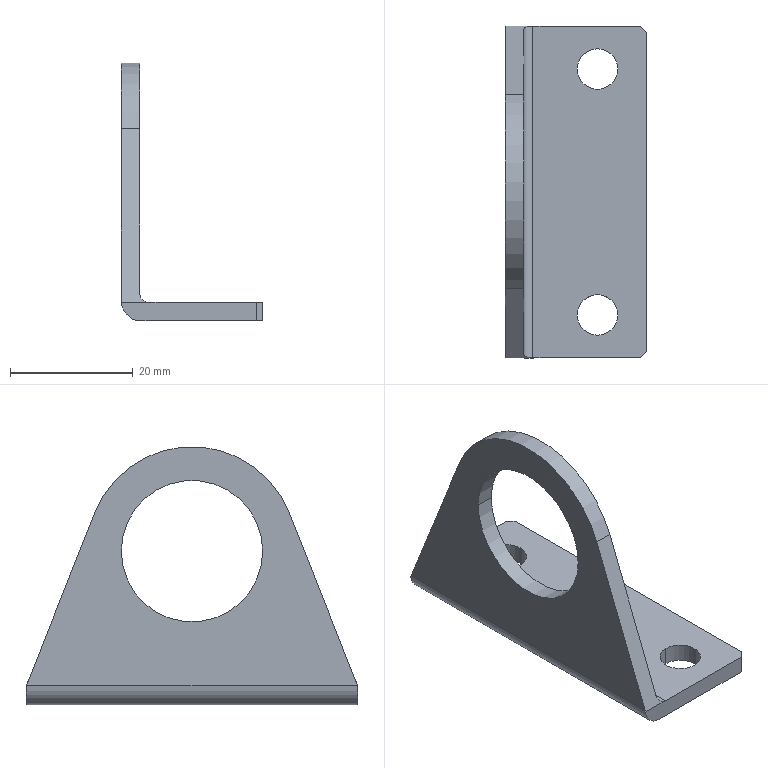Component | SolidWorks | CTM-HVS-42-02-27-1 | 1 solid | 20 faces | box 23 x 54 x 42 mm | volume 6546 mm3 | plane 11 | cylinder 9 | commonest cylinder face diameters 6.6 x4 23 x2 6.4 x1 3 x1 34 x1 | material Q235A Cold Rolled Sheet 3mm
build123d program:
from build123d import *

# Parameters (mm, degrees)
BOSS_EXTRUDE1_DEPTH      = 27
BOSS_EXTRUDE1_DEPTH_BACK = 27
CUT_EXTRUDE1_DEPTH       = 3
CUT_EXTRUDE1_DEPTH_BACK  = 3
SKETCH2_R                = 11.5
CUT_EXTRUDE2_DEPTH       = 6
CUT_EXTRUDE2_DEPTH_BACK  = 6
M6_CLEARANCE_HOLE1_D     = 6.6
CHAMFER1_SIZE            = 1


with BuildPart() as part:
    # Sketch1 → Boss-Extrude1 (new, two sides: drawn at the far end of the back side and taken through both)
    with BuildSketch(Plane.XY.offset(-BOSS_EXTRUDE1_DEPTH_BACK)):
        with BuildLine():
            Line((0, 17), (0, -21.8))
            ThreePointArc((0, -21.8), (0.9373, -24.063), (3.2, -25))
            Line((3.2, -25), (23, -25))
            Line((23, -25), (23, -22))
            Line((23, -22), (4.5, -22))
            ThreePointArc((4.5, -22), (3.439, -21.561), (3, -20.5))
            Line((3, -20.5), (3, 17))
            Line((3, 17), (0, 17))
        make_face()
    extrude(amount=BOSS_EXTRUDE1_DEPTH + BOSS_EXTRUDE1_DEPTH_BACK)

    # Sketch2 → Cut-Extrude1 (cut, two sides: drawn at the far end of the back side and taken through both)
    with BuildSketch(Plane(origin=(0, 0, 0), x_dir=(0, 0, -1), z_dir=(1, 0, 0)).offset(-CUT_EXTRUDE1_DEPTH_BACK)):
        Circle(SKETCH2_R)
    extrude(amount=CUT_EXTRUDE1_DEPTH + CUT_EXTRUDE1_DEPTH_BACK, mode=Mode.SUBTRACT)

    # Sketch3 → Cut-Extrude2 (cut, two sides: drawn at the far end of the back side and taken through both)
    with BuildSketch(Plane(origin=(0, 0, 0), x_dir=(0, 0, -1), z_dir=(1, 0, 0)).offset(-CUT_EXTRUDE2_DEPTH_BACK)):
        with BuildLine():
            Line((-44, -22), (-27, -22))
            Line((-27, -22), (-15.805, 6.261))
            ThreePointArc((-15.805, 6.261), (0, 17), (15.805, 6.261))
            Line((15.805, 6.261), (27, -22))
            Line((27, -22), (44, -22))
            Line((44, -22), (44, 59))
            Line((44, 59), (-44, 59))
            Line((-44, 59), (-44, -22))
        make_face()
    extrude(amount=CUT_EXTRUDE2_DEPTH + CUT_EXTRUDE2_DEPTH_BACK, mode=Mode.SUBTRACT)

    # M6 Clearance Hole1 (through all)
    with Locations(Plane(origin=(0, -22, 0), x_dir=(-1, 0, 0), z_dir=(0, 1, 0))):
        with Locations((-15, 20), (-15, -20)):
            Hole(M6_CLEARANCE_HOLE1_D / 2)

    # Chamfer1
    chamfer1_edges = [part.edges().sort_by_distance(p)[0] for p in [
        (23, -23.5, 27),
        (23, -23.5, -27),
    ]]
    chamfer(chamfer1_edges, length=CHAMFER1_SIZE)


solid = part.part

# Placed as in the assembly
solid = solid.moved(Location((-17.307, 55.443, 30), (90, 0, 0)))
STEP:
#1=CARTESIAN_POINT('',(-0.09084,1.525,0.1969));
#2=VERTEX_POINT('',#1);
#3=CARTESIAN_POINT('',(-0.09084,1.265,0.1969));
#4=VERTEX_POINT('',#3);
#5=CARTESIAN_POINT('',(-0.09084,1.395,0.1969));
#6=DIRECTION('',(0.,0.,1.));
#7=DIRECTION('',(0.,-1.,0.));
#8=AXIS2_PLACEMENT_3D('',#5,#6,#7);
#9=CIRCLE('',#8,0.1299);
#10=EDGE_CURVE('',#2,#4,#9,.T.);
#11=ORIENTED_EDGE('',*,*,#10,.F.);
#12=CARTESIAN_POINT('',(-0.09084,1.525,0.315));
#13=VERTEX_POINT('',#12);
#14=CARTESIAN_POINT('',(-0.09084,1.525,0.315));
#15=DIRECTION('',(0.,0.,1.));
#16=VECTOR('',#15,39.37);
#17=LINE('',#14,#16);
#18=EDGE_CURVE('',#2,#13,#17,.T.);
#19=ORIENTED_EDGE('',*,*,#18,.T.);
#20=CARTESIAN_POINT('',(-0.09084,1.265,0.315));
#21=VERTEX_POINT('',#20);
#22=CARTESIAN_POINT('',(-0.09084,1.395,0.315));
#23=DIRECTION('',(0.,0.,1.));
#24=DIRECTION('',(0.,-1.,0.));
#25=AXIS2_PLACEMENT_3D('',#22,#23,#24);
#26=CIRCLE('',#25,0.1299);
#27=EDGE_CURVE('',#13,#21,#26,.T.);
#28=ORIENTED_EDGE('',*,*,#27,.T.);
#29=CARTESIAN_POINT('',(-0.09084,1.265,0.315));
#30=DIRECTION('',(0.,0.,1.));
#31=VECTOR('',#30,39.37);
#32=LINE('',#29,#31);
#33=EDGE_CURVE('',#4,#21,#32,.T.);
#34=ORIENTED_EDGE('',*,*,#33,.F.);
#35=EDGE_LOOP('',(#11,#19,#28,#34));
#36=FACE_OUTER_BOUND('',#35,.T.);
#37=CARTESIAN_POINT('',(-0.09084,1.395,0.315));
#38=DIRECTION('',(0.,0.,1.));
#39=DIRECTION('',(0.,-1.,0.));
#40=AXIS2_PLACEMENT_3D('',#37,#38,#39);
#41=CYLINDRICAL_SURFACE('',#40,0.1299);
#42=ADVANCED_FACE('',(#36),#41,.F.);
#43=CARTESIAN_POINT('',(-0.09084,3.1,0.1969));
#44=VERTEX_POINT('',#43);
#45=CARTESIAN_POINT('',(-0.09084,2.84,0.1969));
#46=VERTEX_POINT('',#45);
#47=CARTESIAN_POINT('',(-0.09084,2.97,0.1969));
#48=DIRECTION('',(0.,0.,1.));
#49=DIRECTION('',(0.,-1.,0.));
#50=AXIS2_PLACEMENT_3D('',#47,#48,#49);
#51=CIRCLE('',#50,0.1299);
#52=EDGE_CURVE('',#44,#46,#51,.T.);
#53=ORIENTED_EDGE('',*,*,#52,.F.);
#54=CARTESIAN_POINT('',(-0.09084,3.1,0.315));
#55=VERTEX_POINT('',#54);
#56=CARTESIAN_POINT('',(-0.09084,3.1,0.315));
#57=DIRECTION('',(0.,0.,1.));
#58=VECTOR('',#57,39.37);
#59=LINE('',#56,#58);
#60=EDGE_CURVE('',#44,#55,#59,.T.);
#61=ORIENTED_EDGE('',*,*,#60,.T.);
#62=CARTESIAN_POINT('',(-0.09084,2.84,0.315));
#63=VERTEX_POINT('',#62);
#64=CARTESIAN_POINT('',(-0.09084,2.97,0.315));
#65=DIRECTION('',(0.,0.,1.));
#66=DIRECTION('',(0.,-1.,0.));
#67=AXIS2_PLACEMENT_3D('',#64,#65,#66);
#68=CIRCLE('',#67,0.1299);
#69=EDGE_CURVE('',#55,#63,#68,.T.);
#70=ORIENTED_EDGE('',*,*,#69,.T.);
#71=CARTESIAN_POINT('',(-0.09084,2.84,0.315));
#72=DIRECTION('',(0.,0.,1.));
#73=VECTOR('',#72,39.37);
#74=LINE('',#71,#73);
#75=EDGE_CURVE('',#46,#63,#74,.T.);
#76=ORIENTED_EDGE('',*,*,#75,.F.);
#77=EDGE_LOOP('',(#53,#61,#70,#76));
#78=FACE_OUTER_BOUND('',#77,.T.);
#79=CARTESIAN_POINT('',(-0.09084,2.97,0.315));
#80=DIRECTION('',(0.,0.,1.));
#81=DIRECTION('',(0.,-1.,0.));
#82=AXIS2_PLACEMENT_3D('',#79,#80,#81);
#83=CYLINDRICAL_SURFACE('',#82,0.1299);
#84=ADVANCED_FACE('',(#78),#83,.F.);
#85=CARTESIAN_POINT('',(-0.6814,1.73,1.181));
#86=VERTEX_POINT('',#85);
#87=CARTESIAN_POINT('',(-0.6814,2.636,1.181));
#88=VERTEX_POINT('',#87);
#89=CARTESIAN_POINT('',(-0.6814,2.183,1.181));
#90=DIRECTION('',(1.,0.,-0.));
#91=DIRECTION('',(-0.,1.,0.));
#92=AXIS2_PLACEMENT_3D('',#89,#90,#91);
#93=CIRCLE('',#92,0.4528);
#94=EDGE_CURVE('',#86,#88,#93,.T.);
#95=ORIENTED_EDGE('',*,*,#94,.F.);
#96=CARTESIAN_POINT('',(-0.5633,1.73,1.181));
#97=VERTEX_POINT('',#96);
#98=CARTESIAN_POINT('',(-0.7995,1.73,1.181));
#99=DIRECTION('',(1.,0.,-0.));
#100=VECTOR('',#99,39.37);
#101=LINE('',#98,#100);
#102=EDGE_CURVE('',#86,#97,#101,.T.);
#103=ORIENTED_EDGE('',*,*,#102,.T.);
#104=CARTESIAN_POINT('',(-0.5633,2.636,1.181));
#105=VERTEX_POINT('',#104);
#106=CARTESIAN_POINT('',(-0.5633,2.183,1.181));
#107=DIRECTION('',(1.,0.,-0.));
#108=DIRECTION('',(-0.,1.,0.));
#109=AXIS2_PLACEMENT_3D('',#106,#107,#108);
#110=CIRCLE('',#109,0.4528);
#111=EDGE_CURVE('',#97,#105,#110,.T.);
#112=ORIENTED_EDGE('',*,*,#111,.T.);
#113=CARTESIAN_POINT('',(-0.7995,2.636,1.181));
#114=DIRECTION('',(1.,0.,-0.));
#115=VECTOR('',#114,39.37);
#116=LINE('',#113,#115);
#117=EDGE_CURVE('',#88,#105,#116,.T.);
#118=ORIENTED_EDGE('',*,*,#117,.F.);
#119=EDGE_LOOP('',(#95,#103,#112,#118));
#120=FACE_OUTER_BOUND('',#119,.T.);
#121=CARTESIAN_POINT('',(-0.7995,2.183,1.181));
#122=DIRECTION('',(1.,0.,-0.));
#123=DIRECTION('',(-0.,1.,0.));
#124=AXIS2_PLACEMENT_3D('',#121,#122,#123);
#125=CYLINDRICAL_SURFACE('',#124,0.4528);
#126=ADVANCED_FACE('',(#120),#125,.F.);
#127=CARTESIAN_POINT('',(0.2241,1.159,0.315));
#128=VERTEX_POINT('',#127);
#129=CARTESIAN_POINT('',(0.2241,3.206,0.315));
#130=VERTEX_POINT('',#129);
#131=CARTESIAN_POINT('',(0.2241,1.12,0.315));
#132=DIRECTION('',(-0.,1.,-0.));
#133=VECTOR('',#132,39.37);
#134=LINE('',#131,#133);
#135=EDGE_CURVE('',#128,#130,#134,.T.);
#136=ORIENTED_EDGE('',*,*,#135,.T.);
#137=CARTESIAN_POINT('',(0.1848,3.246,0.315));
#138=VERTEX_POINT('',#137);
#139=CARTESIAN_POINT('',(0.2241,3.206,0.315));
#140=DIRECTION('',(-0.7071,0.7071,-0.));
#141=VECTOR('',#140,39.37);
#142=LINE('',#139,#141);
#143=EDGE_CURVE('',#130,#138,#142,.T.);
#144=ORIENTED_EDGE('',*,*,#143,.T.);
#145=CARTESIAN_POINT('',(-0.5042,3.246,0.315));
#146=VERTEX_POINT('',#145);
#147=CARTESIAN_POINT('',(0.2241,3.246,0.315));
#148=DIRECTION('',(-1.,-0.,0.));
#149=VECTOR('',#148,39.37);
#150=LINE('',#147,#149);
#151=EDGE_CURVE('',#138,#146,#150,.T.);
#152=ORIENTED_EDGE('',*,*,#151,.T.);
#153=CARTESIAN_POINT('',(-0.5042,1.12,0.315));
#154=VERTEX_POINT('',#153);
#155=CARTESIAN_POINT('',(-0.5042,1.12,0.315));
#156=DIRECTION('',(-0.,1.,-0.));
#157=VECTOR('',#156,39.37);
#158=LINE('',#155,#157);
#159=EDGE_CURVE('',#154,#146,#158,.T.);
#160=ORIENTED_EDGE('',*,*,#159,.F.);
#161=CARTESIAN_POINT('',(0.1848,1.12,0.315));
#162=VERTEX_POINT('',#161);
#163=CARTESIAN_POINT('',(0.2241,1.12,0.315));
#164=DIRECTION('',(-1.,-0.,0.));
#165=VECTOR('',#164,39.37);
#166=LINE('',#163,#165);
#167=EDGE_CURVE('',#162,#154,#166,.T.);
#168=ORIENTED_EDGE('',*,*,#167,.F.);
#169=CARTESIAN_POINT('',(0.1848,1.12,0.315));
#170=DIRECTION('',(0.7071,0.7071,-0.));
#171=VECTOR('',#170,39.37);
#172=LINE('',#169,#171);
#173=EDGE_CURVE('',#162,#128,#172,.T.);
#174=ORIENTED_EDGE('',*,*,#173,.T.);
#175=EDGE_LOOP('',(#136,#144,#152,#160,#168,#174));
#176=FACE_OUTER_BOUND('',#175,.T.);
#177=CARTESIAN_POINT('',(-0.09084,2.97,0.315));
#178=DIRECTION('',(0.,0.,1.));
#179=DIRECTION('',(0.,-1.,0.));
#180=AXIS2_PLACEMENT_3D('',#177,#178,#179);
#181=CIRCLE('',#180,0.1299);
#182=EDGE_CURVE('',#63,#55,#181,.T.);
#183=ORIENTED_EDGE('',*,*,#182,.F.);
#184=ORIENTED_EDGE('',*,*,#69,.F.);
#185=EDGE_LOOP('',(#183,#184));
#186=FACE_BOUND('',#185,.T.);
#187=CARTESIAN_POINT('',(-0.09084,1.395,0.315));
#188=DIRECTION('',(0.,0.,1.));
#189=DIRECTION('',(0.,-1.,0.));
#190=AXIS2_PLACEMENT_3D('',#187,#188,#189);
#191=CIRCLE('',#190,0.1299);
#192=EDGE_CURVE('',#21,#13,#191,.T.);
#193=ORIENTED_EDGE('',*,*,#192,.F.);
#194=ORIENTED_EDGE('',*,*,#27,.F.);
#195=EDGE_LOOP('',(#193,#194));
#196=FACE_BOUND('',#195,.T.);
#197=CARTESIAN_POINT('',(0.2241,1.12,0.315));
#198=DIRECTION('',(-0.,-0.,-1.));
#199=DIRECTION('',(-0.,1.,-0.));
#200=AXIS2_PLACEMENT_3D('',#197,#198,#199);
#201=PLANE('',#200);
#202=ADVANCED_FACE('',(#176,#186,#196),#201,.F.);
#203=CARTESIAN_POINT('',(-0.6814,2.183,1.181));
#204=DIRECTION('',(1.,0.,-0.));
#205=DIRECTION('',(-0.,1.,0.));
#206=AXIS2_PLACEMENT_3D('',#203,#204,#205);
#207=CIRCLE('',#206,0.4528);
#208=EDGE_CURVE('',#88,#86,#207,.T.);
#209=ORIENTED_EDGE('',*,*,#208,.T.);
#210=ORIENTED_EDGE('',*,*,#94,.T.);
#211=EDGE_LOOP('',(#209,#210));
#212=FACE_BOUND('',#211,.T.);
#213=CARTESIAN_POINT('',(-0.6814,1.561,1.428));
#214=VERTEX_POINT('',#213);
#215=CARTESIAN_POINT('',(-0.6814,2.805,1.428));
#216=VERTEX_POINT('',#215);
#217=CARTESIAN_POINT('',(-0.6814,2.183,1.181));
#218=DIRECTION('',(-1.,-0.,0.));
#219=DIRECTION('',(-0.,1.,0.));
#220=AXIS2_PLACEMENT_3D('',#217,#218,#219);
#221=CIRCLE('',#220,0.6693);
#222=EDGE_CURVE('',#214,#216,#221,.T.);
#223=ORIENTED_EDGE('',*,*,#222,.T.);
#224=CARTESIAN_POINT('',(-0.6814,3.243,0.3228));
#225=VERTEX_POINT('',#224);
#226=CARTESIAN_POINT('',(-0.6814,2.432,2.37));
#227=DIRECTION('',(-0.,0.3683,-0.9297));
#228=VECTOR('',#227,39.37);
#229=LINE('',#226,#228);
#230=EDGE_CURVE('',#216,#225,#229,.T.);
#231=ORIENTED_EDGE('',*,*,#230,.T.);
#232=CARTESIAN_POINT('',(-0.6814,1.123,0.3228));
#233=VERTEX_POINT('',#232);
#234=CARTESIAN_POINT('',(-0.6814,1.12,0.3228));
#235=DIRECTION('',(-0.,1.,-0.));
#236=VECTOR('',#235,39.37);
#237=LINE('',#234,#236);
#238=EDGE_CURVE('',#233,#225,#237,.T.);
#239=ORIENTED_EDGE('',*,*,#238,.F.);
#240=CARTESIAN_POINT('',(-0.6814,1.646,1.642));
#241=DIRECTION('',(-0.,0.3683,0.9297));
#242=VECTOR('',#241,39.37);
#243=LINE('',#240,#242);
#244=EDGE_CURVE('',#233,#214,#243,.T.);
#245=ORIENTED_EDGE('',*,*,#244,.T.);
#246=EDGE_LOOP('',(#223,#231,#239,#245));
#247=FACE_OUTER_BOUND('',#246,.T.);
#248=CARTESIAN_POINT('',(-0.6814,1.12,1.85));
#249=DIRECTION('',(1.,0.,-0.));
#250=DIRECTION('',(-0.,1.,-0.));
#251=AXIS2_PLACEMENT_3D('',#248,#249,#250);
#252=PLANE('',#251);
#253=ADVANCED_FACE('',(#212,#247),#252,.F.);
#254=ORIENTED_EDGE('',*,*,#238,.T.);
#255=CARTESIAN_POINT('',(-0.6811,3.246,0.315));
#256=VERTEX_POINT('',#255);
#257=CARTESIAN_POINT('',(-0.6814,3.243,0.3228));
#258=CARTESIAN_POINT('',(-0.6814,3.244,0.3202));
#259=CARTESIAN_POINT('',(-0.6813,3.245,0.3176));
#260=CARTESIAN_POINT('',(-0.6811,3.246,0.315));
#261=(BOUNDED_CURVE()B_SPLINE_CURVE(3,(#257,#258,#259,#260),.UNSPECIFIED.,.F.,.F.)B_SPLINE_CURVE_WITH_KNOTS((4,4),(4.712,4.775),.UNSPECIFIED.)CURVE()GEOMETRIC_REPRESENTATION_ITEM()RATIONAL_B_SPLINE_CURVE((1.,0.9997,0.9997,1.))REPRESENTATION_ITEM(''));
#262=EDGE_CURVE('',#225,#256,#261,.T.);
#263=ORIENTED_EDGE('',*,*,#262,.T.);
#264=CARTESIAN_POINT('',(-0.5554,3.246,0.1969));
#265=VERTEX_POINT('',#264);
#266=CARTESIAN_POINT('',(-0.5554,3.246,0.3228));
#267=DIRECTION('',(0.,-1.,0.));
#268=DIRECTION('',(1.,0.,0.));
#269=AXIS2_PLACEMENT_3D('',#266,#267,#268);
#270=CIRCLE('',#269,0.126);
#271=EDGE_CURVE('',#256,#265,#270,.T.);
#272=ORIENTED_EDGE('',*,*,#271,.T.);
#273=CARTESIAN_POINT('',(-0.5554,1.12,0.1969));
#274=VERTEX_POINT('',#273);
#275=CARTESIAN_POINT('',(-0.5554,1.12,0.1969));
#276=DIRECTION('',(-0.,1.,-0.));
#277=VECTOR('',#276,39.37);
#278=LINE('',#275,#277);
#279=EDGE_CURVE('',#274,#265,#278,.T.);
#280=ORIENTED_EDGE('',*,*,#279,.F.);
#281=CARTESIAN_POINT('',(-0.6811,1.12,0.315));
#282=VERTEX_POINT('',#281);
#283=CARTESIAN_POINT('',(-0.5554,1.12,0.3228));
#284=DIRECTION('',(0.,-1.,0.));
#285=DIRECTION('',(1.,0.,0.));
#286=AXIS2_PLACEMENT_3D('',#283,#284,#285);
#287=CIRCLE('',#286,0.126);
#288=EDGE_CURVE('',#282,#274,#287,.T.);
#289=ORIENTED_EDGE('',*,*,#288,.F.);
#290=CARTESIAN_POINT('',(-0.6811,1.12,0.315));
#291=CARTESIAN_POINT('',(-0.6813,1.121,0.3176));
#292=CARTESIAN_POINT('',(-0.6814,1.122,0.3202));
#293=CARTESIAN_POINT('',(-0.6814,1.123,0.3228));
#294=(BOUNDED_CURVE()B_SPLINE_CURVE(3,(#290,#291,#292,#293),.UNSPECIFIED.,.F.,.T.)B_SPLINE_CURVE_WITH_KNOTS((4,4),(4.65,4.712),.UNSPECIFIED.)CURVE()GEOMETRIC_REPRESENTATION_ITEM()RATIONAL_B_SPLINE_CURVE((1.,0.9997,0.9997,1.))REPRESENTATION_ITEM(''));
#295=EDGE_CURVE('',#282,#233,#294,.T.);
#296=ORIENTED_EDGE('',*,*,#295,.T.);
#297=EDGE_LOOP('',(#254,#263,#272,#280,#289,#296));
#298=FACE_OUTER_BOUND('',#297,.T.);
#299=CARTESIAN_POINT('',(-0.5554,1.12,0.3228));
#300=DIRECTION('',(-0.,1.,-0.));
#301=DIRECTION('',(-1.,-0.,0.));
#302=AXIS2_PLACEMENT_3D('',#299,#300,#301);
#303=CYLINDRICAL_SURFACE('',#302,0.126);
#304=ADVANCED_FACE('',(#298),#303,.T.);
#305=CARTESIAN_POINT('',(-0.09084,1.395,0.1969));
#306=DIRECTION('',(0.,0.,1.));
#307=DIRECTION('',(0.,-1.,0.));
#308=AXIS2_PLACEMENT_3D('',#305,#306,#307);
#309=CIRCLE('',#308,0.1299);
#310=EDGE_CURVE('',#4,#2,#309,.T.);
#311=ORIENTED_EDGE('',*,*,#310,.T.);
#312=ORIENTED_EDGE('',*,*,#10,.T.);
#313=EDGE_LOOP('',(#311,#312));
#314=FACE_BOUND('',#313,.T.);
#315=CARTESIAN_POINT('',(-0.09084,2.97,0.1969));
#316=DIRECTION('',(0.,0.,1.));
#317=DIRECTION('',(0.,-1.,0.));
#318=AXIS2_PLACEMENT_3D('',#315,#316,#317);
#319=CIRCLE('',#318,0.1299);
#320=EDGE_CURVE('',#46,#44,#319,.T.);
#321=ORIENTED_EDGE('',*,*,#320,.T.);
#322=ORIENTED_EDGE('',*,*,#52,.T.);
#323=EDGE_LOOP('',(#321,#322));
#324=FACE_BOUND('',#323,.T.);
#325=CARTESIAN_POINT('',(0.1848,3.246,0.1969));
#326=VERTEX_POINT('',#325);
#327=CARTESIAN_POINT('',(-0.5554,3.246,0.1969));
#328=DIRECTION('',(1.,0.,-0.));
#329=VECTOR('',#328,39.37);
#330=LINE('',#327,#329);
#331=EDGE_CURVE('',#265,#326,#330,.T.);
#332=ORIENTED_EDGE('',*,*,#331,.T.);
#333=CARTESIAN_POINT('',(0.2241,3.206,0.1969));
#334=VERTEX_POINT('',#333);
#335=CARTESIAN_POINT('',(0.2241,3.206,0.1969));
#336=DIRECTION('',(0.7071,-0.7071,0.));
#337=VECTOR('',#336,39.37);
#338=LINE('',#335,#337);
#339=EDGE_CURVE('',#326,#334,#338,.T.);
#340=ORIENTED_EDGE('',*,*,#339,.T.);
#341=CARTESIAN_POINT('',(0.2241,1.159,0.1969));
#342=VERTEX_POINT('',#341);
#343=CARTESIAN_POINT('',(0.2241,1.12,0.1969));
#344=DIRECTION('',(-0.,1.,-0.));
#345=VECTOR('',#344,39.37);
#346=LINE('',#343,#345);
#347=EDGE_CURVE('',#342,#334,#346,.T.);
#348=ORIENTED_EDGE('',*,*,#347,.F.);
#349=CARTESIAN_POINT('',(0.1848,1.12,0.1969));
#350=VERTEX_POINT('',#349);
#351=CARTESIAN_POINT('',(0.1848,1.12,0.1969));
#352=DIRECTION('',(-0.7071,-0.7071,0.));
#353=VECTOR('',#352,39.37);
#354=LINE('',#351,#353);
#355=EDGE_CURVE('',#342,#350,#354,.T.);
#356=ORIENTED_EDGE('',*,*,#355,.T.);
#357=CARTESIAN_POINT('',(-0.5554,1.12,0.1969));
#358=DIRECTION('',(1.,0.,-0.));
#359=VECTOR('',#358,39.37);
#360=LINE('',#357,#359);
#361=EDGE_CURVE('',#274,#350,#360,.T.);
#362=ORIENTED_EDGE('',*,*,#361,.F.);
#363=ORIENTED_EDGE('',*,*,#279,.T.);
#364=EDGE_LOOP('',(#332,#340,#348,#356,#362,#363));
#365=FACE_OUTER_BOUND('',#364,.T.);
#366=CARTESIAN_POINT('',(-0.5554,1.12,0.1969));
#367=DIRECTION('',(0.,0.,1.));
#368=DIRECTION('',(0.,-1.,0.));
#369=AXIS2_PLACEMENT_3D('',#366,#367,#368);
#370=PLANE('',#369);
#371=ADVANCED_FACE('',(#314,#324,#365),#370,.F.);
#372=ORIENTED_EDGE('',*,*,#347,.T.);
#373=CARTESIAN_POINT('',(0.2241,3.206,0.1969));
#374=DIRECTION('',(0.,0.,1.));
#375=VECTOR('',#374,39.37);
#376=LINE('',#373,#375);
#377=EDGE_CURVE('',#334,#130,#376,.T.);
#378=ORIENTED_EDGE('',*,*,#377,.T.);
#379=ORIENTED_EDGE('',*,*,#135,.F.);
#380=CARTESIAN_POINT('',(0.2241,1.159,0.1969));
#381=DIRECTION('',(-0.,-0.,-1.));
#382=VECTOR('',#381,39.37);
#383=LINE('',#380,#382);
#384=EDGE_CURVE('',#128,#342,#383,.T.);
#385=ORIENTED_EDGE('',*,*,#384,.T.);
#386=EDGE_LOOP('',(#372,#378,#379,#385));
#387=FACE_OUTER_BOUND('',#386,.T.);
#388=CARTESIAN_POINT('',(0.2241,1.12,0.1969));
#389=DIRECTION('',(-1.,-0.,0.));
#390=DIRECTION('',(0.,-1.,0.));
#391=AXIS2_PLACEMENT_3D('',#388,#389,#390);
#392=PLANE('',#391);
#393=ADVANCED_FACE('',(#387),#392,.F.);
#394=ORIENTED_EDGE('',*,*,#159,.T.);
#395=CARTESIAN_POINT('',(-0.5633,3.222,0.374));
#396=VERTEX_POINT('',#395);
#397=CARTESIAN_POINT('',(-0.5042,3.246,0.315));
#398=CARTESIAN_POINT('',(-0.5388,3.246,0.315));
#399=CARTESIAN_POINT('',(-0.5633,3.236,0.3394));
#400=CARTESIAN_POINT('',(-0.5633,3.222,0.374));
#401=(BOUNDED_CURVE()B_SPLINE_CURVE(3,(#397,#398,#399,#400),.UNSPECIFIED.,.F.,.T.)B_SPLINE_CURVE_WITH_KNOTS((4,4),(0.,1.571),.UNSPECIFIED.)CURVE()GEOMETRIC_REPRESENTATION_ITEM()RATIONAL_B_SPLINE_CURVE((1.,0.8047,0.8047,1.))REPRESENTATION_ITEM(''));
#402=EDGE_CURVE('',#146,#396,#401,.T.);
#403=ORIENTED_EDGE('',*,*,#402,.T.);
#404=CARTESIAN_POINT('',(-0.5633,1.143,0.374));
#405=VERTEX_POINT('',#404);
#406=CARTESIAN_POINT('',(-0.5633,1.12,0.374));
#407=DIRECTION('',(-0.,1.,-0.));
#408=VECTOR('',#407,39.37);
#409=LINE('',#406,#408);
#410=EDGE_CURVE('',#405,#396,#409,.T.);
#411=ORIENTED_EDGE('',*,*,#410,.F.);
#412=CARTESIAN_POINT('',(-0.5633,1.143,0.374));
#413=CARTESIAN_POINT('',(-0.5633,1.129,0.3394));
#414=CARTESIAN_POINT('',(-0.5388,1.12,0.315));
#415=CARTESIAN_POINT('',(-0.5042,1.12,0.315));
#416=(BOUNDED_CURVE()B_SPLINE_CURVE(3,(#412,#413,#414,#415),.UNSPECIFIED.,.F.,.F.)B_SPLINE_CURVE_WITH_KNOTS((4,4),(1.571,3.142),.UNSPECIFIED.)CURVE()GEOMETRIC_REPRESENTATION_ITEM()RATIONAL_B_SPLINE_CURVE((1.,0.8047,0.8047,1.))REPRESENTATION_ITEM(''));
#417=EDGE_CURVE('',#405,#154,#416,.T.);
#418=ORIENTED_EDGE('',*,*,#417,.T.);
#419=EDGE_LOOP('',(#394,#403,#411,#418));
#420=FACE_OUTER_BOUND('',#419,.T.);
#421=CARTESIAN_POINT('',(-0.5042,1.12,0.374));
#422=DIRECTION('',(-0.,1.,-0.));
#423=DIRECTION('',(-1.,-0.,0.));
#424=AXIS2_PLACEMENT_3D('',#421,#422,#423);
#425=CYLINDRICAL_SURFACE('',#424,0.05906);
#426=ADVANCED_FACE('',(#420),#425,.F.);
#427=CARTESIAN_POINT('',(-0.5633,2.183,1.181));
#428=DIRECTION('',(1.,0.,-0.));
#429=DIRECTION('',(-0.,1.,0.));
#430=AXIS2_PLACEMENT_3D('',#427,#428,#429);
#431=CIRCLE('',#430,0.4528);
#432=EDGE_CURVE('',#105,#97,#431,.T.);
#433=ORIENTED_EDGE('',*,*,#432,.F.);
#434=ORIENTED_EDGE('',*,*,#111,.F.);
#435=EDGE_LOOP('',(#433,#434));
#436=FACE_BOUND('',#435,.T.);
#437=ORIENTED_EDGE('',*,*,#410,.T.);
#438=CARTESIAN_POINT('',(-0.5633,2.805,1.428));
#439=VERTEX_POINT('',#438);
#440=CARTESIAN_POINT('',(-0.5633,2.937,1.094));
#441=DIRECTION('',(0.,-0.3683,0.9297));
#442=VECTOR('',#441,39.37);
#443=LINE('',#440,#442);
#444=EDGE_CURVE('',#396,#439,#443,.T.);
#445=ORIENTED_EDGE('',*,*,#444,.T.);
#446=CARTESIAN_POINT('',(-0.5633,1.561,1.428));
#447=VERTEX_POINT('',#446);
#448=CARTESIAN_POINT('',(-0.5633,2.183,1.181));
#449=DIRECTION('',(1.,0.,-0.));
#450=DIRECTION('',(0.,-1.,0.));
#451=AXIS2_PLACEMENT_3D('',#448,#449,#450);
#452=CIRCLE('',#451,0.6693);
#453=EDGE_CURVE('',#439,#447,#452,.T.);
#454=ORIENTED_EDGE('',*,*,#453,.T.);
#455=CARTESIAN_POINT('',(-0.5633,1.14,0.366));
#456=DIRECTION('',(0.,-0.3683,-0.9297));
#457=VECTOR('',#456,39.37);
#458=LINE('',#455,#457);
#459=EDGE_CURVE('',#447,#405,#458,.T.);
#460=ORIENTED_EDGE('',*,*,#459,.T.);
#461=EDGE_LOOP('',(#437,#445,#454,#460));
#462=FACE_OUTER_BOUND('',#461,.T.);
#463=CARTESIAN_POINT('',(-0.5633,1.12,0.374));
#464=DIRECTION('',(-1.,-0.,0.));
#465=DIRECTION('',(0.,-1.,0.));
#466=AXIS2_PLACEMENT_3D('',#463,#464,#465);
#467=PLANE('',#466);
#468=ADVANCED_FACE('',(#436,#462),#467,.F.);
#469=ORIENTED_EDGE('',*,*,#361,.T.);
#470=CARTESIAN_POINT('',(0.1848,1.12,0.315));
#471=DIRECTION('',(0.,0.,1.));
#472=VECTOR('',#471,39.37);
#473=LINE('',#470,#472);
#474=EDGE_CURVE('',#350,#162,#473,.T.);
#475=ORIENTED_EDGE('',*,*,#474,.T.);
#476=ORIENTED_EDGE('',*,*,#167,.T.);
#477=CARTESIAN_POINT('',(-0.5554,1.12,0.315));
#478=DIRECTION('',(1.,0.,-0.));
#479=VECTOR('',#478,39.37);
#480=LINE('',#477,#479);
#481=EDGE_CURVE('',#282,#154,#480,.T.);
#482=ORIENTED_EDGE('',*,*,#481,.F.);
#483=ORIENTED_EDGE('',*,*,#288,.T.);
#484=EDGE_LOOP('',(#469,#475,#476,#482,#483));
#485=FACE_OUTER_BOUND('',#484,.T.);
#486=CARTESIAN_POINT('',(-0.5554,1.12,0.3228));
#487=DIRECTION('',(0.,-1.,0.));
#488=DIRECTION('',(1.,0.,-0.));
#489=AXIS2_PLACEMENT_3D('',#486,#487,#488);
#490=PLANE('',#489);
#491=ADVANCED_FACE('',(#485),#490,.T.);
#492=ORIENTED_EDGE('',*,*,#151,.F.);
#493=CARTESIAN_POINT('',(0.1848,3.246,0.3228));
#494=DIRECTION('',(-0.,-0.,-1.));
#495=VECTOR('',#494,39.37);
#496=LINE('',#493,#495);
#497=EDGE_CURVE('',#138,#326,#496,.T.);
#498=ORIENTED_EDGE('',*,*,#497,.T.);
#499=ORIENTED_EDGE('',*,*,#331,.F.);
#500=ORIENTED_EDGE('',*,*,#271,.F.);
#501=CARTESIAN_POINT('',(-0.5554,3.246,0.315));
#502=DIRECTION('',(1.,0.,-0.));
#503=VECTOR('',#502,39.37);
#504=LINE('',#501,#503);
#505=EDGE_CURVE('',#256,#146,#504,.T.);
#506=ORIENTED_EDGE('',*,*,#505,.T.);
#507=EDGE_LOOP('',(#492,#498,#499,#500,#506));
#508=FACE_OUTER_BOUND('',#507,.T.);
#509=CARTESIAN_POINT('',(-0.5554,3.246,0.3228));
#510=DIRECTION('',(0.,-1.,0.));
#511=DIRECTION('',(1.,0.,-0.));
#512=AXIS2_PLACEMENT_3D('',#509,#510,#511);
#513=PLANE('',#512);
#514=ADVANCED_FACE('',(#508),#513,.F.);
#515=ORIENTED_EDGE('',*,*,#102,.F.);
#516=ORIENTED_EDGE('',*,*,#208,.F.);
#517=ORIENTED_EDGE('',*,*,#117,.T.);
#518=ORIENTED_EDGE('',*,*,#432,.T.);
#519=EDGE_LOOP('',(#515,#516,#517,#518));
#520=FACE_OUTER_BOUND('',#519,.T.);
#521=CARTESIAN_POINT('',(-0.7995,2.183,1.181));
#522=DIRECTION('',(1.,0.,-0.));
#523=DIRECTION('',(-0.,1.,0.));
#524=AXIS2_PLACEMENT_3D('',#521,#522,#523);
#525=CYLINDRICAL_SURFACE('',#524,0.4528);
#526=ADVANCED_FACE('',(#520),#525,.F.);
#527=ORIENTED_EDGE('',*,*,#453,.F.);
#528=CARTESIAN_POINT('',(-0.9176,2.805,1.428));
#529=DIRECTION('',(1.,0.,-0.));
#530=VECTOR('',#529,39.37);
#531=LINE('',#528,#530);
#532=EDGE_CURVE('',#216,#439,#531,.T.);
#533=ORIENTED_EDGE('',*,*,#532,.F.);
#534=ORIENTED_EDGE('',*,*,#222,.F.);
#535=CARTESIAN_POINT('',(-0.9176,1.561,1.428));
#536=DIRECTION('',(1.,0.,-0.));
#537=VECTOR('',#536,39.37);
#538=LINE('',#535,#537);
#539=EDGE_CURVE('',#214,#447,#538,.T.);
#540=ORIENTED_EDGE('',*,*,#539,.T.);
#541=EDGE_LOOP('',(#527,#533,#534,#540));
#542=FACE_OUTER_BOUND('',#541,.T.);
#543=CARTESIAN_POINT('',(-0.9176,2.183,1.181));
#544=DIRECTION('',(1.,0.,-0.));
#545=DIRECTION('',(-0.,1.,0.));
#546=AXIS2_PLACEMENT_3D('',#543,#544,#545);
#547=CYLINDRICAL_SURFACE('',#546,0.6693);
#548=ADVANCED_FACE('',(#542),#547,.T.);
#549=ORIENTED_EDGE('',*,*,#295,.F.);
#550=ORIENTED_EDGE('',*,*,#481,.T.);
#551=ORIENTED_EDGE('',*,*,#417,.F.);
#552=ORIENTED_EDGE('',*,*,#459,.F.);
#553=ORIENTED_EDGE('',*,*,#539,.F.);
#554=ORIENTED_EDGE('',*,*,#244,.F.);
#555=EDGE_LOOP('',(#549,#550,#551,#552,#553,#554));
#556=FACE_OUTER_BOUND('',#555,.T.);
#557=CARTESIAN_POINT('',(-0.9176,1.12,0.315));
#558=DIRECTION('',(-0.,0.9297,-0.3683));
#559=DIRECTION('',(-0.,0.3683,0.9297));
#560=AXIS2_PLACEMENT_3D('',#557,#558,#559);
#561=PLANE('',#560);
#562=ADVANCED_FACE('',(#556),#561,.F.);
#563=ORIENTED_EDGE('',*,*,#532,.T.);
#564=ORIENTED_EDGE('',*,*,#444,.F.);
#565=ORIENTED_EDGE('',*,*,#402,.F.);
#566=ORIENTED_EDGE('',*,*,#505,.F.);
#567=ORIENTED_EDGE('',*,*,#262,.F.);
#568=ORIENTED_EDGE('',*,*,#230,.F.);
#569=EDGE_LOOP('',(#563,#564,#565,#566,#567,#568));
#570=FACE_OUTER_BOUND('',#569,.T.);
#571=CARTESIAN_POINT('',(-0.9176,2.805,1.428));
#572=DIRECTION('',(0.,-0.9297,-0.3683));
#573=DIRECTION('',(-0.,0.3683,-0.9297));
#574=AXIS2_PLACEMENT_3D('',#571,#572,#573);
#575=PLANE('',#574);
#576=ADVANCED_FACE('',(#570),#575,.F.);
#577=ORIENTED_EDGE('',*,*,#60,.F.);
#578=ORIENTED_EDGE('',*,*,#320,.F.);
#579=ORIENTED_EDGE('',*,*,#75,.T.);
#580=ORIENTED_EDGE('',*,*,#182,.T.);
#581=EDGE_LOOP('',(#577,#578,#579,#580));
#582=FACE_OUTER_BOUND('',#581,.T.);
#583=CARTESIAN_POINT('',(-0.09084,2.97,0.315));
#584=DIRECTION('',(0.,0.,1.));
#585=DIRECTION('',(0.,-1.,0.));
#586=AXIS2_PLACEMENT_3D('',#583,#584,#585);
#587=CYLINDRICAL_SURFACE('',#586,0.1299);
#588=ADVANCED_FACE('',(#582),#587,.F.);
#589=ORIENTED_EDGE('',*,*,#18,.F.);
#590=ORIENTED_EDGE('',*,*,#310,.F.);
#591=ORIENTED_EDGE('',*,*,#33,.T.);
#592=ORIENTED_EDGE('',*,*,#192,.T.);
#593=EDGE_LOOP('',(#589,#590,#591,#592));
#594=FACE_OUTER_BOUND('',#593,.T.);
#595=CARTESIAN_POINT('',(-0.09084,1.395,0.315));
#596=DIRECTION('',(0.,0.,1.));
#597=DIRECTION('',(0.,-1.,0.));
#598=AXIS2_PLACEMENT_3D('',#595,#596,#597);
#599=CYLINDRICAL_SURFACE('',#598,0.1299);
#600=ADVANCED_FACE('',(#594),#599,.F.);
#601=ORIENTED_EDGE('',*,*,#339,.F.);
#602=ORIENTED_EDGE('',*,*,#497,.F.);
#603=ORIENTED_EDGE('',*,*,#143,.F.);
#604=ORIENTED_EDGE('',*,*,#377,.F.);
#605=EDGE_LOOP('',(#601,#602,#603,#604));
#606=FACE_OUTER_BOUND('',#605,.T.);
#607=CARTESIAN_POINT('',(0.2241,3.206,0.1969));
#608=DIRECTION('',(-0.7071,-0.7071,0.));
#609=DIRECTION('',(0.7071,-0.7071,0.));
#610=AXIS2_PLACEMENT_3D('',#607,#608,#609);
#611=PLANE('',#610);
#612=ADVANCED_FACE('',(#606),#611,.F.);
#613=ORIENTED_EDGE('',*,*,#355,.F.);
#614=ORIENTED_EDGE('',*,*,#384,.F.);
#615=ORIENTED_EDGE('',*,*,#173,.F.);
#616=ORIENTED_EDGE('',*,*,#474,.F.);
#617=EDGE_LOOP('',(#613,#614,#615,#616));
#618=FACE_OUTER_BOUND('',#617,.T.);
#619=CARTESIAN_POINT('',(0.1848,1.12,0.3228));
#620=DIRECTION('',(0.7071,-0.7071,0.));
#621=DIRECTION('',(0.7071,0.7071,-0.));
#622=AXIS2_PLACEMENT_3D('',#619,#620,#621);
#623=PLANE('',#622);
#624=ADVANCED_FACE('',(#618),#623,.T.);
#625=CLOSED_SHELL('',(#42,#84,#126,#202,#253,#304,#371,#393,#426,#468,#491,#514,#526,#548,#562,#576,#588,#600,#612,#624));
#626=MANIFOLD_SOLID_BREP('',#625);
#627=CARTESIAN_POINT('',(0.,0.,0.));
#628=DIRECTION('',(0.,0.,1.));
#629=DIRECTION('',(1.,0.,0.));
#630=AXIS2_PLACEMENT_3D('',#627,#628,#629);
#631=(LENGTH_UNIT()NAMED_UNIT(*)SI_UNIT($,.METRE.));
#632=LENGTH_MEASURE_WITH_UNIT(LENGTH_MEASURE(0.0254),#631);
#633=DIMENSIONAL_EXPONENTS(1.,0.,0.,0.,0.,0.,0.);
#634=(CONVERSION_BASED_UNIT('',#632)LENGTH_UNIT()NAMED_UNIT(#633));
#635=UNCERTAINTY_MEASURE_WITH_UNIT(LENGTH_MEASURE(0.00001),#634,'','');
#636=(NAMED_UNIT(*)PLANE_ANGLE_UNIT()SI_UNIT($,.RADIAN.));
#637=(NAMED_UNIT(*)SI_UNIT($,.STERADIAN.)SOLID_ANGLE_UNIT());
#638=(GEOMETRIC_REPRESENTATION_CONTEXT(3)GLOBAL_UNCERTAINTY_ASSIGNED_CONTEXT((#635))GLOBAL_UNIT_ASSIGNED_CONTEXT((#634,#636,#637))REPRESENTATION_CONTEXT('',''));
#639=ADVANCED_BREP_SHAPE_REPRESENTATION('',(#626,#630),#638);
#640=COLOUR_RGB('',0.7922,0.8196,0.9333);
#641=FILL_AREA_STYLE_COLOUR('',#640);
#642=FILL_AREA_STYLE('',(#641));
#643=SURFACE_STYLE_FILL_AREA(#642);
#644=SURFACE_SIDE_STYLE('',(#643));
#645=SURFACE_STYLE_USAGE(.BOTH.,#644);
#646=PRESENTATION_STYLE_ASSIGNMENT((#645));
#647=STYLED_ITEM('',(#646),#626);
#648=PRESENTATION_LAYER_ASSIGNMENT('','',(#647));
#649=(LENGTH_UNIT()NAMED_UNIT(*)SI_UNIT($,.METRE.));
#650=LENGTH_MEASURE_WITH_UNIT(LENGTH_MEASURE(0.0254),#649);
#651=DIMENSIONAL_EXPONENTS(1.,0.,0.,0.,0.,0.,0.);
#652=(CONVERSION_BASED_UNIT('',#650)LENGTH_UNIT()NAMED_UNIT(#651));
#653=UNCERTAINTY_MEASURE_WITH_UNIT(LENGTH_MEASURE(0.00001),#652,'','');
#654=(NAMED_UNIT(*)PLANE_ANGLE_UNIT()SI_UNIT($,.RADIAN.));
#655=(NAMED_UNIT(*)SI_UNIT($,.STERADIAN.)SOLID_ANGLE_UNIT());
#656=(GEOMETRIC_REPRESENTATION_CONTEXT(3)GLOBAL_UNCERTAINTY_ASSIGNED_CONTEXT((#653))GLOBAL_UNIT_ASSIGNED_CONTEXT((#652,#654,#655))REPRESENTATION_CONTEXT('',''));
#657=MECHANICAL_DESIGN_GEOMETRIC_PRESENTATION_REPRESENTATION('',(#647),#656);